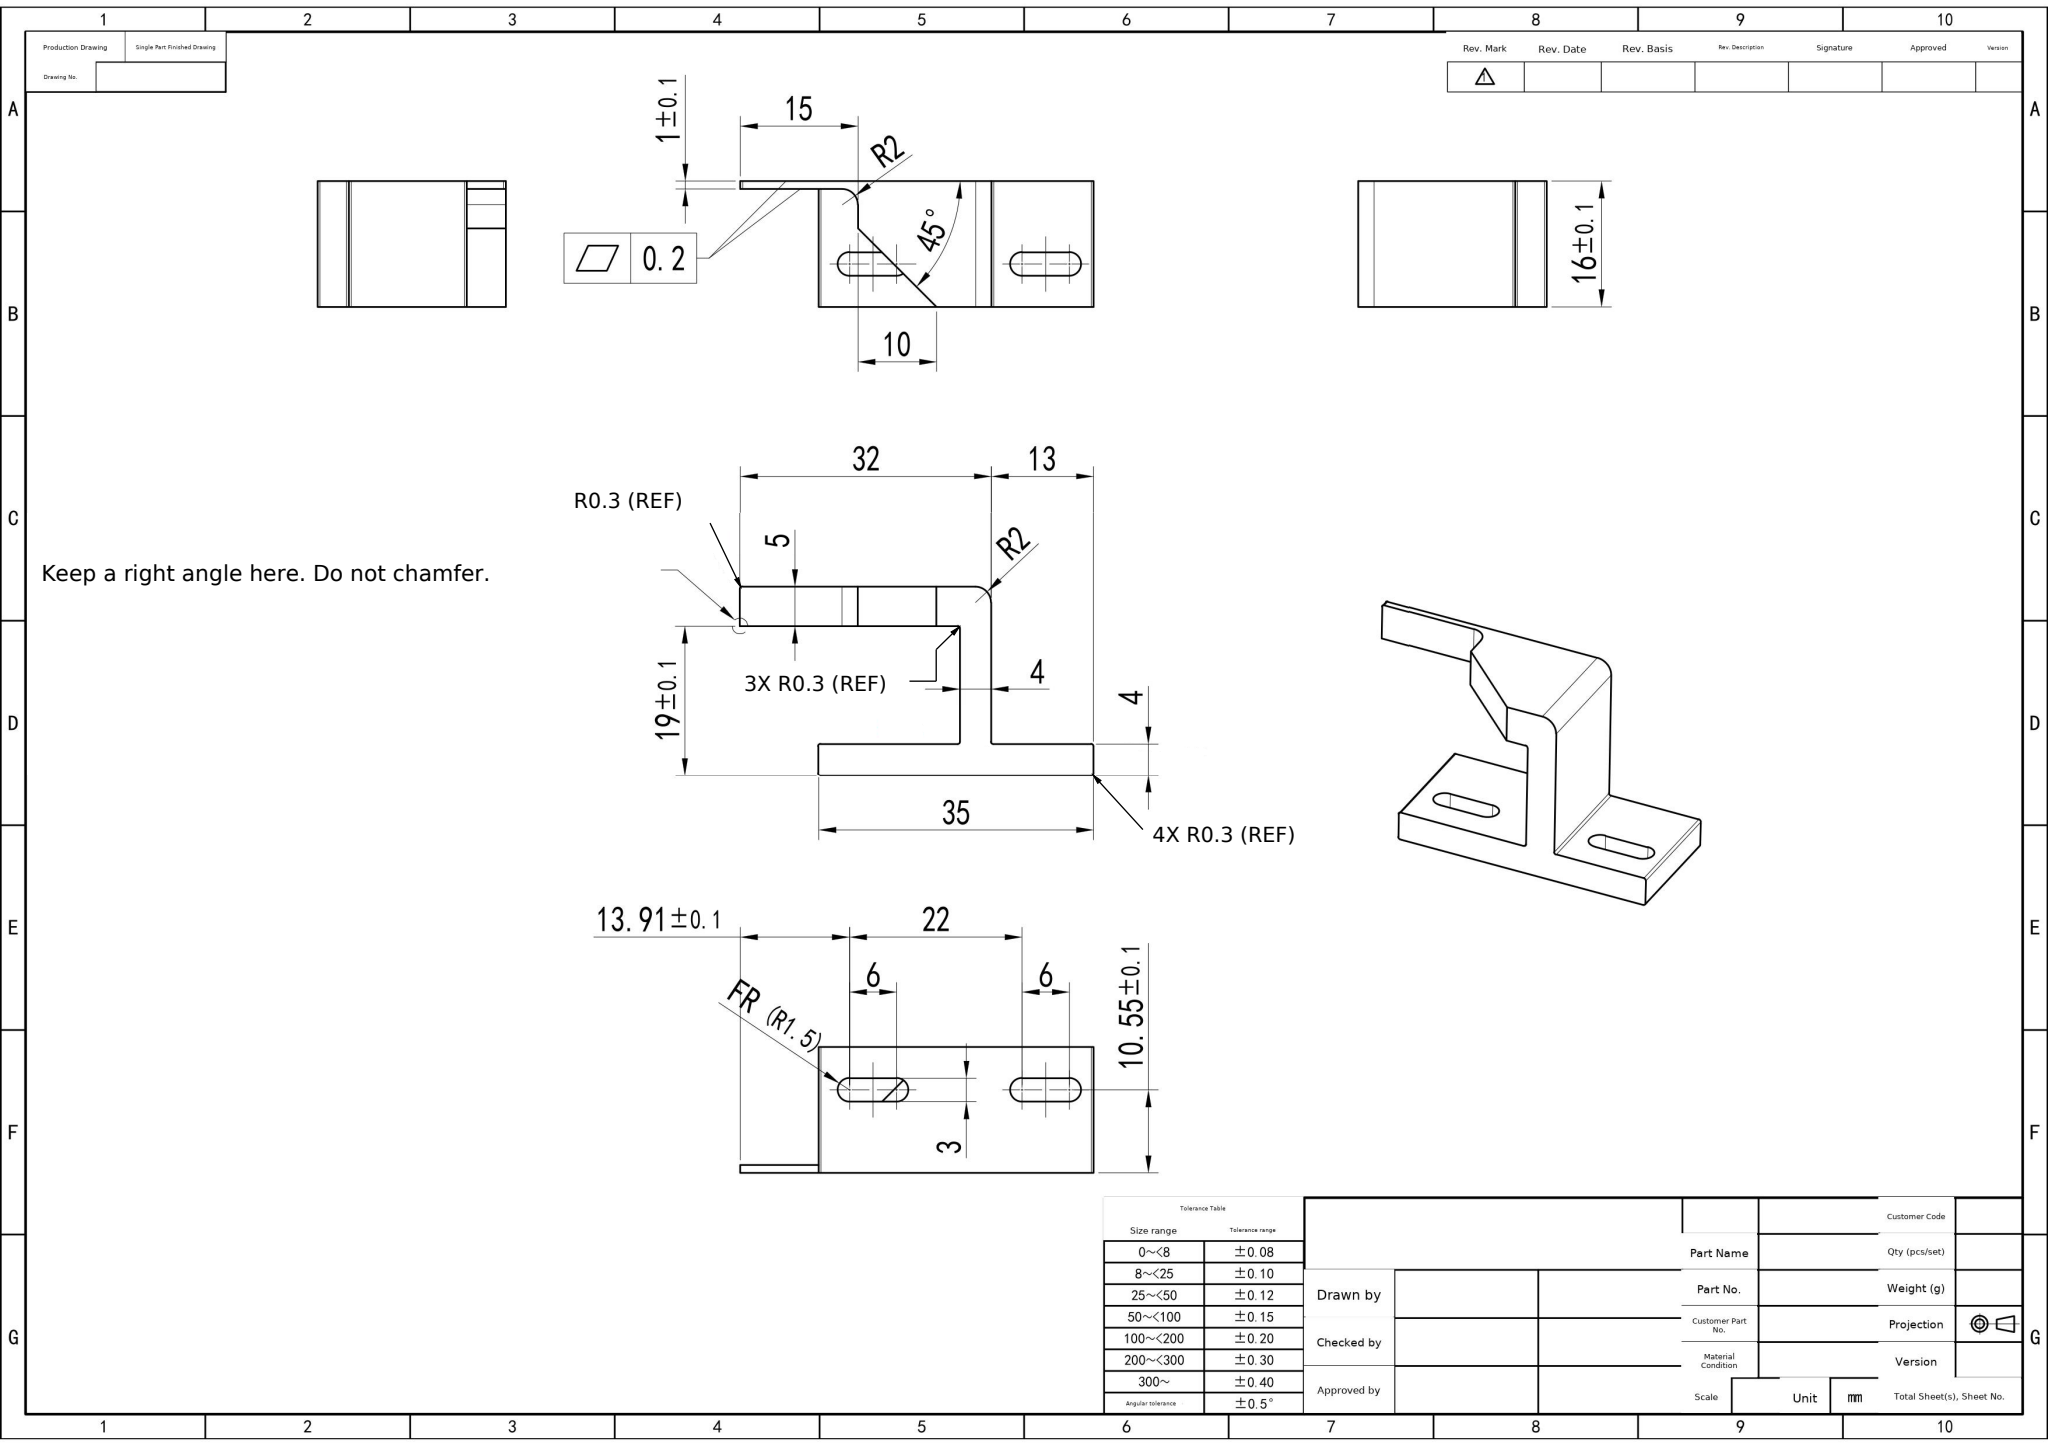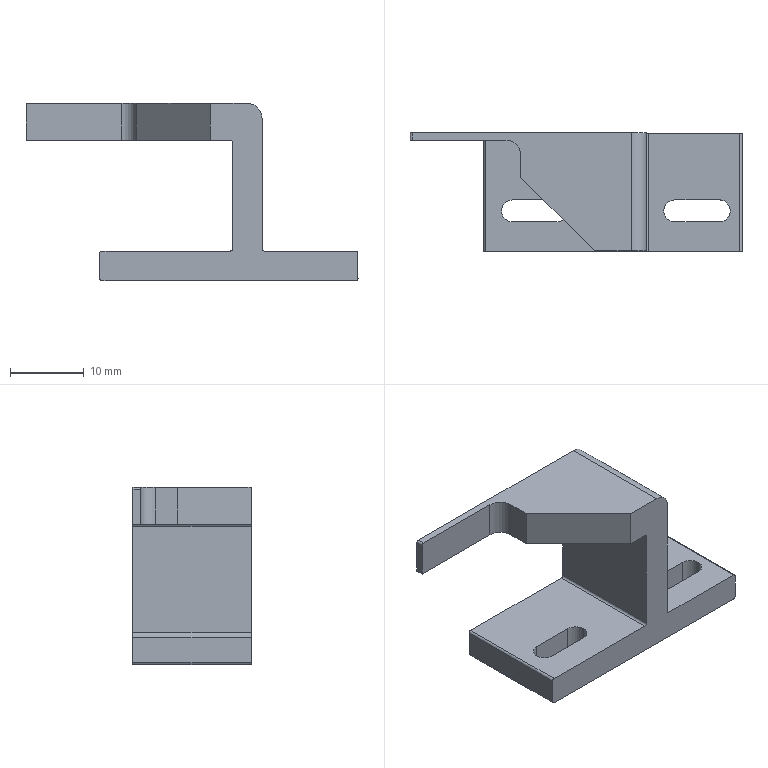Part | SolidWorks | mm | 1 solid | 35 faces | box 45 x 16 x 24 mm | volume 4175 mm3 | plane 19 | cylinder 16 | commonest cylinder face diameters 0.6 x8 3 x6 4 x2